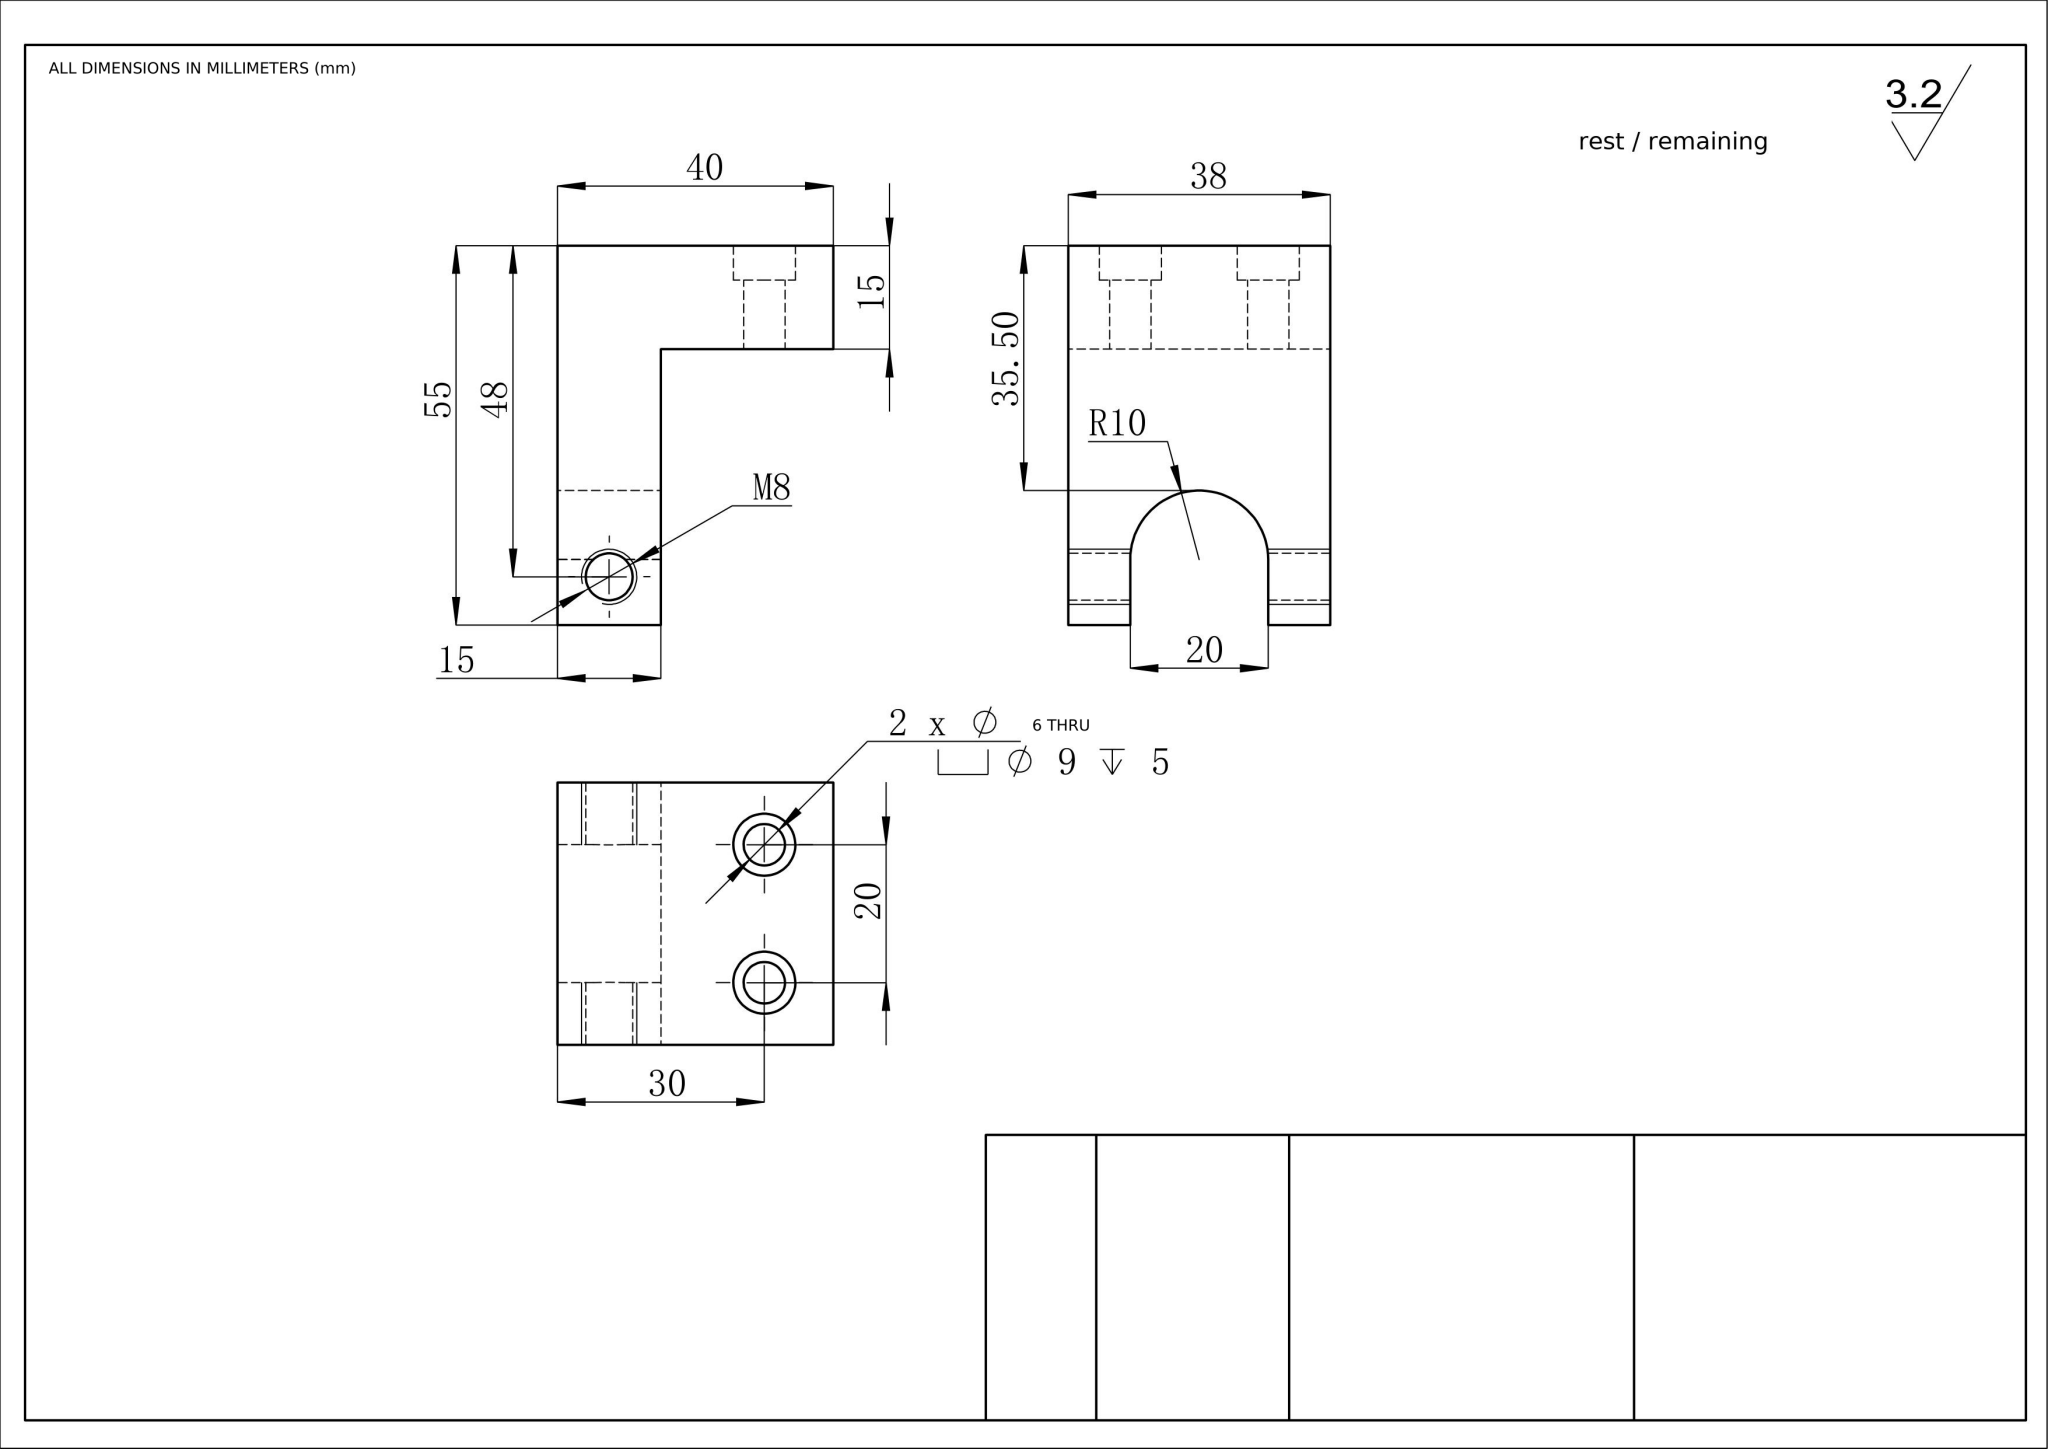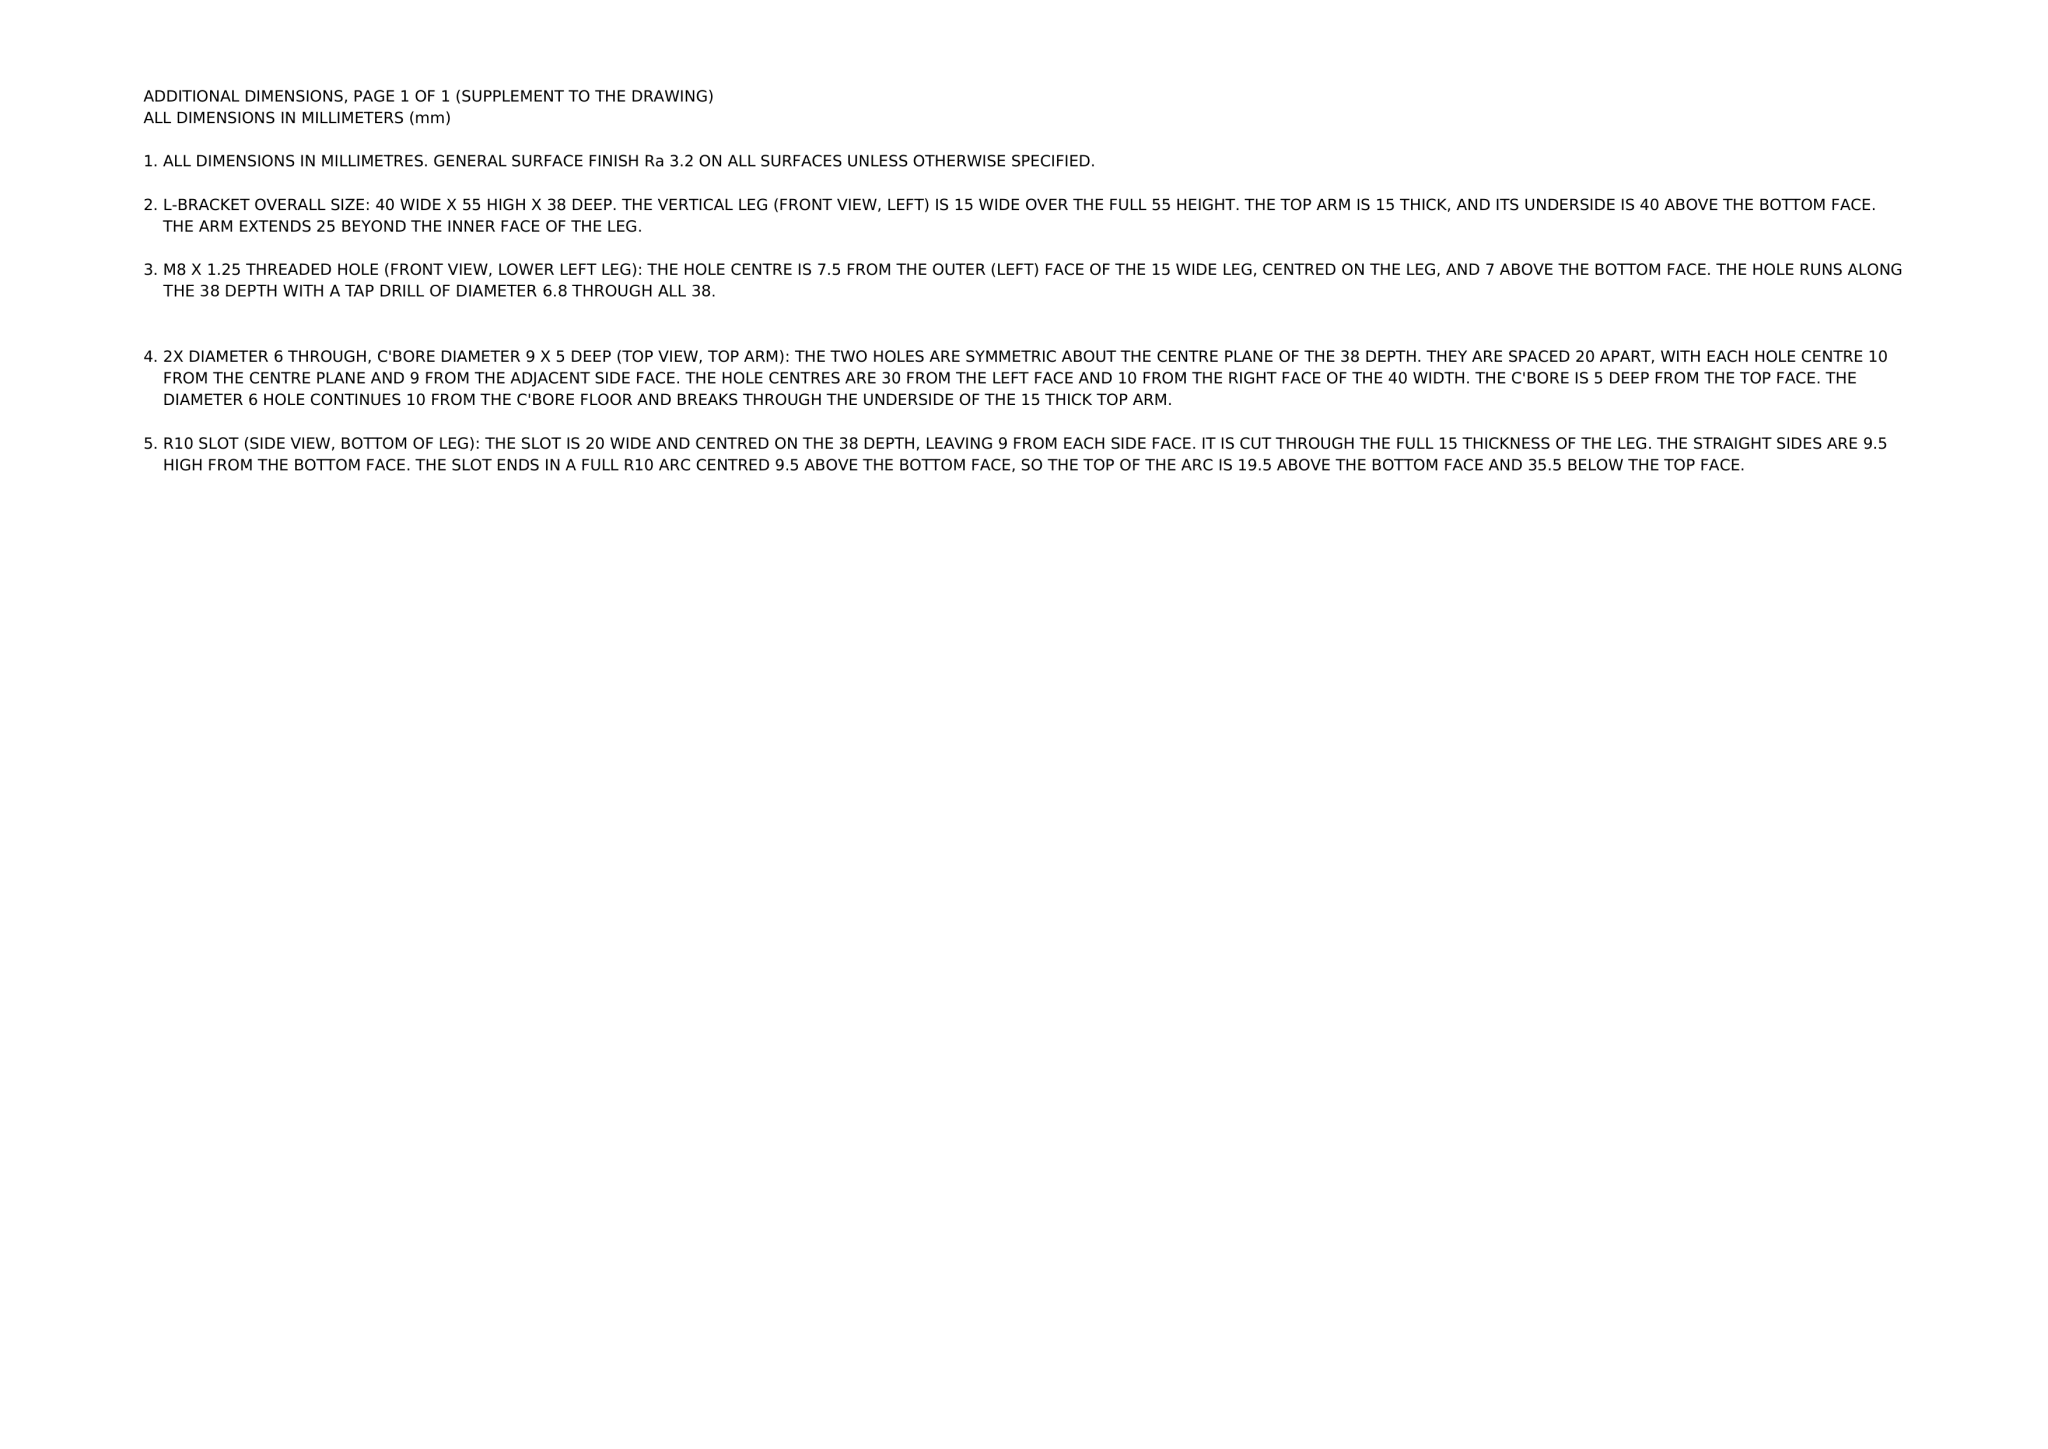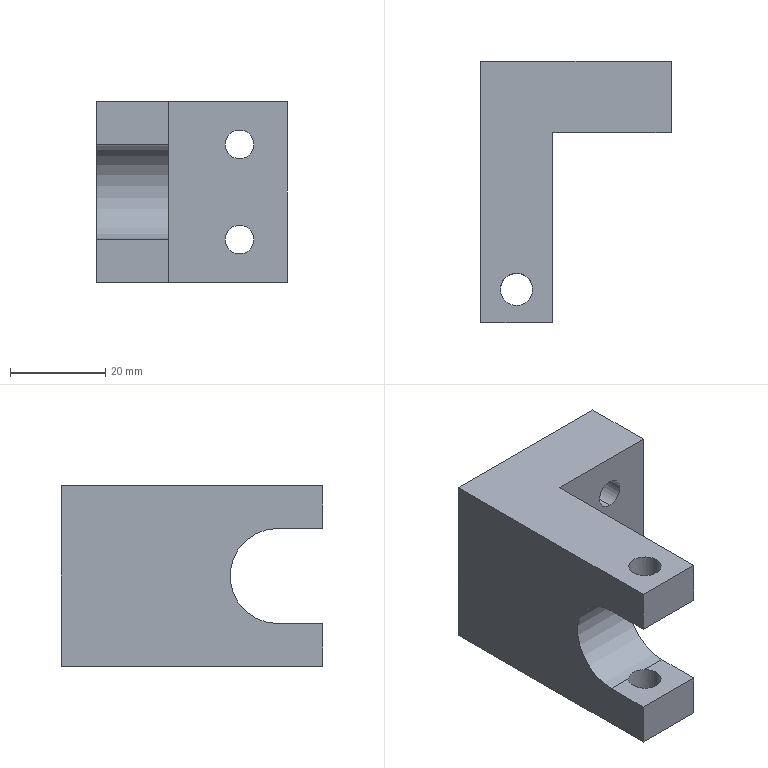Part | NX | mm | 1 solid | 26 faces | box 40 x 55 x 38 mm | volume 38538 mm3 | cylinder 13 | plane 13 | commonest cylinder face diameters 9 x4 6 x4 6.8 x4 20 x1